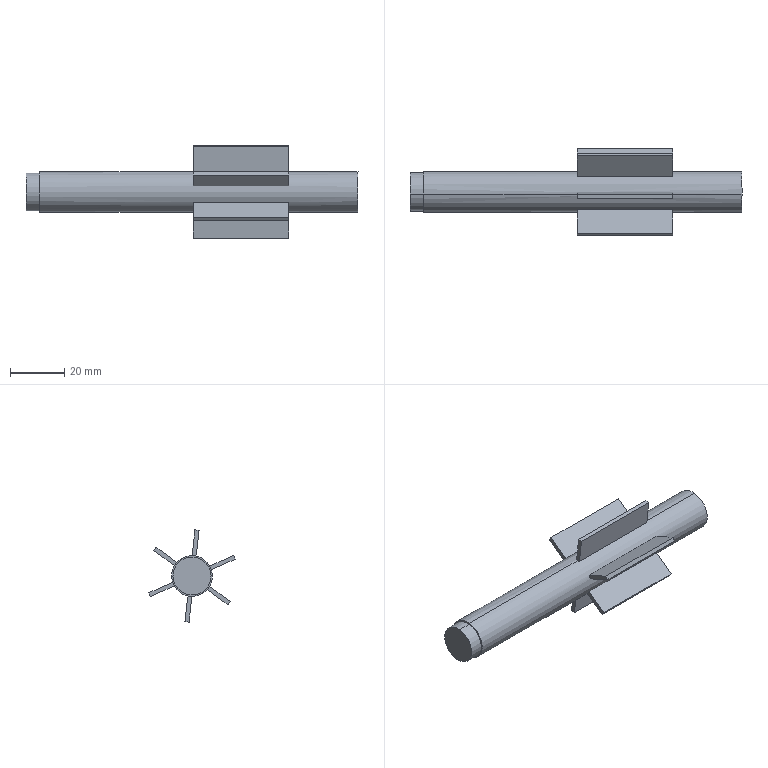Component | SolidWorks | HZ022-A001-E004-1 | 1 solid | 37 faces | box 122 x 31.71 x 33.96 mm | volume 24441 mm3 | plane 33 | cylinder 4 | commonest cylinder face diameters 13.99 x2 15 x2 | material S45C
STEP:
#1=COLOUR_RGB('',0.7922,0.8196,0.9333);
#2=FILL_AREA_STYLE_COLOUR('',#1);
#3=FILL_AREA_STYLE('',(#2));
#4=SURFACE_STYLE_FILL_AREA(#3);
#5=SURFACE_SIDE_STYLE('',(#4));
#6=SURFACE_STYLE_USAGE(.BOTH.,#5);
#7=PRESENTATION_STYLE_ASSIGNMENT((#6));
#8=CARTESIAN_POINT('',(-1.518,7.595,35.553));
#9=VERTEX_POINT('',#8);
#10=CARTESIAN_POINT('',(-1.518,7.535,36.101));
#11=VERTEX_POINT('',#10);
#12=CARTESIAN_POINT('',(-1.518,7.565,35.827));
#13=DIRECTION('',(1.,-0.,-0.));
#14=DIRECTION('',(-0.,0.108,-0.9942));
#15=AXIS2_PLACEMENT_3D('',#12,#13,#14);
#16=CIRCLE('',#15,0.2754);
#17=EDGE_CURVE('',#9,#11,#16,.T.);
#18=ORIENTED_EDGE('',*,*,#17,.F.);
#19=CARTESIAN_POINT('',(-1.715,7.595,35.553));
#20=VERTEX_POINT('',#19);
#21=CARTESIAN_POINT('',(-1.518,7.595,35.553));
#22=DIRECTION('',(-1.,0.,0.));
#23=VECTOR('',#22,39.37);
#24=LINE('',#21,#23);
#25=EDGE_CURVE('',#9,#20,#24,.T.);
#26=ORIENTED_EDGE('',*,*,#25,.T.);
#27=CARTESIAN_POINT('',(-1.715,7.535,36.101));
#28=VERTEX_POINT('',#27);
#29=CARTESIAN_POINT('',(-1.715,7.565,35.827));
#30=DIRECTION('',(-1.,0.,0.));
#31=DIRECTION('',(-0.,0.108,-0.9942));
#32=AXIS2_PLACEMENT_3D('',#29,#30,#31);
#33=CIRCLE('',#32,0.2754);
#34=EDGE_CURVE('',#28,#20,#33,.T.);
#35=ORIENTED_EDGE('',*,*,#34,.F.);
#36=CARTESIAN_POINT('',(-1.518,7.535,36.101));
#37=DIRECTION('',(-1.,0.,0.));
#38=VECTOR('',#37,39.37);
#39=LINE('',#36,#38);
#40=EDGE_CURVE('',#11,#28,#39,.T.);
#41=ORIENTED_EDGE('',*,*,#40,.F.);
#42=EDGE_LOOP('',(#18,#26,#35,#41));
#43=FACE_OUTER_BOUND('',#42,.T.);
#44=CARTESIAN_POINT('',(-1.518,7.565,35.827));
#45=DIRECTION('',(-1.,0.,0.));
#46=DIRECTION('',(0.,-0.108,0.9942));
#47=AXIS2_PLACEMENT_3D('',#44,#45,#46);
#48=CYLINDRICAL_SURFACE('',#47,0.2754);
#49=ADVANCED_FACE('',(#43),#48,.T.);
#50=CARTESIAN_POINT('',(2.084,7.785,36.024));
#51=VERTEX_POINT('',#50);
#52=CARTESIAN_POINT('',(2.084,7.82,35.976));
#53=VERTEX_POINT('',#52);
#54=CARTESIAN_POINT('',(2.084,7.565,35.827));
#55=DIRECTION('',(-1.,0.,0.));
#56=DIRECTION('',(0.,-0.108,0.9942));
#57=AXIS2_PLACEMENT_3D('',#54,#55,#56);
#58=CIRCLE('',#57,0.2953);
#59=EDGE_CURVE('',#51,#53,#58,.T.);
#60=ORIENTED_EDGE('',*,*,#59,.F.);
#61=CARTESIAN_POINT('',(0.7064,7.785,36.024));
#62=VERTEX_POINT('',#61);
#63=CARTESIAN_POINT('',(3.088,7.785,36.024));
#64=DIRECTION('',(-1.,0.,0.));
#65=VECTOR('',#64,39.37);
#66=LINE('',#63,#65);
#67=EDGE_CURVE('',#51,#62,#66,.T.);
#68=ORIENTED_EDGE('',*,*,#67,.T.);
#69=CARTESIAN_POINT('',(0.7064,7.82,35.976));
#70=VERTEX_POINT('',#69);
#71=CARTESIAN_POINT('',(0.7064,7.565,35.827));
#72=DIRECTION('',(-1.,0.,0.));
#73=DIRECTION('',(0.,-0.108,0.9942));
#74=AXIS2_PLACEMENT_3D('',#71,#72,#73);
#75=CIRCLE('',#74,0.2953);
#76=EDGE_CURVE('',#62,#70,#75,.T.);
#77=ORIENTED_EDGE('',*,*,#76,.T.);
#78=CARTESIAN_POINT('',(3.088,7.82,35.976));
#79=DIRECTION('',(1.,-0.,-0.));
#80=VECTOR('',#79,39.37);
#81=LINE('',#78,#80);
#82=EDGE_CURVE('',#70,#53,#81,.T.);
#83=ORIENTED_EDGE('',*,*,#82,.T.);
#84=EDGE_LOOP('',(#60,#68,#77,#83));
#85=FACE_BOUND('',#84,.T.);
#86=CARTESIAN_POINT('',(0.7064,7.846,35.735));
#87=VERTEX_POINT('',#86);
#88=CARTESIAN_POINT('',(0.7064,7.822,35.681));
#89=VERTEX_POINT('',#88);
#90=CARTESIAN_POINT('',(0.7064,7.565,35.827));
#91=DIRECTION('',(-1.,0.,0.));
#92=DIRECTION('',(0.,-0.108,0.9942));
#93=AXIS2_PLACEMENT_3D('',#90,#91,#92);
#94=CIRCLE('',#93,0.2953);
#95=EDGE_CURVE('',#87,#89,#94,.T.);
#96=ORIENTED_EDGE('',*,*,#95,.T.);
#97=CARTESIAN_POINT('',(2.084,7.822,35.681));
#98=VERTEX_POINT('',#97);
#99=CARTESIAN_POINT('',(3.088,7.822,35.681));
#100=DIRECTION('',(1.,-0.,-0.));
#101=VECTOR('',#100,39.37);
#102=LINE('',#99,#101);
#103=EDGE_CURVE('',#89,#98,#102,.T.);
#104=ORIENTED_EDGE('',*,*,#103,.T.);
#105=CARTESIAN_POINT('',(2.084,7.846,35.735));
#106=VERTEX_POINT('',#105);
#107=CARTESIAN_POINT('',(2.084,7.565,35.827));
#108=DIRECTION('',(-1.,0.,0.));
#109=DIRECTION('',(0.,-0.108,0.9942));
#110=AXIS2_PLACEMENT_3D('',#107,#108,#109);
#111=CIRCLE('',#110,0.2953);
#112=EDGE_CURVE('',#106,#98,#111,.T.);
#113=ORIENTED_EDGE('',*,*,#112,.F.);
#114=CARTESIAN_POINT('',(3.088,7.846,35.735));
#115=DIRECTION('',(1.,-0.,-0.));
#116=VECTOR('',#115,39.37);
#117=LINE('',#114,#116);
#118=EDGE_CURVE('',#87,#106,#117,.T.);
#119=ORIENTED_EDGE('',*,*,#118,.F.);
#120=EDGE_LOOP('',(#96,#104,#113,#119));
#121=FACE_BOUND('',#120,.T.);
#122=CARTESIAN_POINT('',(3.088,7.597,35.533));
#123=VERTEX_POINT('',#122);
#124=CARTESIAN_POINT('',(3.088,7.533,36.12));
#125=VERTEX_POINT('',#124);
#126=CARTESIAN_POINT('',(3.088,7.565,35.827));
#127=DIRECTION('',(1.,-0.,-0.));
#128=DIRECTION('',(-0.,0.108,-0.9942));
#129=AXIS2_PLACEMENT_3D('',#126,#127,#128);
#130=CIRCLE('',#129,0.2953);
#131=EDGE_CURVE('',#123,#125,#130,.T.);
#132=ORIENTED_EDGE('',*,*,#131,.F.);
#133=CARTESIAN_POINT('',(2.084,7.597,35.533));
#134=VERTEX_POINT('',#133);
#135=CARTESIAN_POINT('',(3.088,7.597,35.533));
#136=DIRECTION('',(-1.,0.,0.));
#137=VECTOR('',#136,39.37);
#138=LINE('',#135,#137);
#139=EDGE_CURVE('',#123,#134,#138,.T.);
#140=ORIENTED_EDGE('',*,*,#139,.T.);
#141=CARTESIAN_POINT('',(2.084,7.626,35.538));
#142=VERTEX_POINT('',#141);
#143=CARTESIAN_POINT('',(2.084,7.565,35.827));
#144=DIRECTION('',(-1.,0.,0.));
#145=DIRECTION('',(0.,-0.108,0.9942));
#146=AXIS2_PLACEMENT_3D('',#143,#144,#145);
#147=CIRCLE('',#146,0.2953);
#148=EDGE_CURVE('',#142,#134,#147,.T.);
#149=ORIENTED_EDGE('',*,*,#148,.F.);
#150=CARTESIAN_POINT('',(0.7064,7.626,35.538));
#151=VERTEX_POINT('',#150);
#152=CARTESIAN_POINT('',(3.088,7.626,35.538));
#153=DIRECTION('',(1.,-0.,-0.));
#154=VECTOR('',#153,39.37);
#155=LINE('',#152,#154);
#156=EDGE_CURVE('',#151,#142,#155,.T.);
#157=ORIENTED_EDGE('',*,*,#156,.F.);
#158=CARTESIAN_POINT('',(0.7064,7.597,35.533));
#159=VERTEX_POINT('',#158);
#160=CARTESIAN_POINT('',(0.7064,7.565,35.827));
#161=DIRECTION('',(-1.,0.,0.));
#162=DIRECTION('',(0.,-0.108,0.9942));
#163=AXIS2_PLACEMENT_3D('',#160,#161,#162);
#164=CIRCLE('',#163,0.2953);
#165=EDGE_CURVE('',#151,#159,#164,.T.);
#166=ORIENTED_EDGE('',*,*,#165,.T.);
#167=CARTESIAN_POINT('',(-1.518,7.597,35.533));
#168=VERTEX_POINT('',#167);
#169=CARTESIAN_POINT('',(3.088,7.597,35.533));
#170=DIRECTION('',(-1.,0.,0.));
#171=VECTOR('',#170,39.37);
#172=LINE('',#169,#171);
#173=EDGE_CURVE('',#159,#168,#172,.T.);
#174=ORIENTED_EDGE('',*,*,#173,.T.);
#175=CARTESIAN_POINT('',(-1.518,7.533,36.12));
#176=VERTEX_POINT('',#175);
#177=CARTESIAN_POINT('',(-1.518,7.565,35.827));
#178=DIRECTION('',(1.,-0.,-0.));
#179=DIRECTION('',(-0.,0.108,-0.9942));
#180=AXIS2_PLACEMENT_3D('',#177,#178,#179);
#181=CIRCLE('',#180,0.2953);
#182=EDGE_CURVE('',#168,#176,#181,.T.);
#183=ORIENTED_EDGE('',*,*,#182,.T.);
#184=CARTESIAN_POINT('',(0.7064,7.533,36.12));
#185=VERTEX_POINT('',#184);
#186=CARTESIAN_POINT('',(3.088,7.533,36.12));
#187=DIRECTION('',(-1.,0.,0.));
#188=VECTOR('',#187,39.37);
#189=LINE('',#186,#188);
#190=EDGE_CURVE('',#185,#176,#189,.T.);
#191=ORIENTED_EDGE('',*,*,#190,.F.);
#192=CARTESIAN_POINT('',(0.7064,7.563,36.122));
#193=VERTEX_POINT('',#192);
#194=CARTESIAN_POINT('',(0.7064,7.565,35.827));
#195=DIRECTION('',(-1.,0.,0.));
#196=DIRECTION('',(0.,-0.108,0.9942));
#197=AXIS2_PLACEMENT_3D('',#194,#195,#196);
#198=CIRCLE('',#197,0.2953);
#199=EDGE_CURVE('',#185,#193,#198,.T.);
#200=ORIENTED_EDGE('',*,*,#199,.T.);
#201=CARTESIAN_POINT('',(2.084,7.563,36.122));
#202=VERTEX_POINT('',#201);
#203=CARTESIAN_POINT('',(3.088,7.563,36.122));
#204=DIRECTION('',(1.,-0.,-0.));
#205=VECTOR('',#204,39.37);
#206=LINE('',#203,#205);
#207=EDGE_CURVE('',#193,#202,#206,.T.);
#208=ORIENTED_EDGE('',*,*,#207,.T.);
#209=CARTESIAN_POINT('',(2.084,7.533,36.12));
#210=VERTEX_POINT('',#209);
#211=CARTESIAN_POINT('',(2.084,7.565,35.827));
#212=DIRECTION('',(-1.,0.,0.));
#213=DIRECTION('',(0.,-0.108,0.9942));
#214=AXIS2_PLACEMENT_3D('',#211,#212,#213);
#215=CIRCLE('',#214,0.2953);
#216=EDGE_CURVE('',#210,#202,#215,.T.);
#217=ORIENTED_EDGE('',*,*,#216,.F.);
#218=CARTESIAN_POINT('',(3.088,7.533,36.12));
#219=DIRECTION('',(-1.,0.,0.));
#220=VECTOR('',#219,39.37);
#221=LINE('',#218,#220);
#222=EDGE_CURVE('',#125,#210,#221,.T.);
#223=ORIENTED_EDGE('',*,*,#222,.F.);
#224=EDGE_LOOP('',(#132,#140,#149,#157,#166,#174,#183,#191,#200,#208,#217,#223));
#225=FACE_OUTER_BOUND('',#224,.T.);
#226=CARTESIAN_POINT('',(3.088,7.565,35.827));
#227=DIRECTION('',(-1.,0.,0.));
#228=DIRECTION('',(0.,-0.108,0.9942));
#229=AXIS2_PLACEMENT_3D('',#226,#227,#228);
#230=CYLINDRICAL_SURFACE('',#229,0.2953);
#231=ADVANCED_FACE('',(#85,#121,#225),#230,.T.);
#232=ORIENTED_EDGE('',*,*,#139,.F.);
#233=CARTESIAN_POINT('',(3.088,7.565,35.827));
#234=DIRECTION('',(1.,-0.,-0.));
#235=DIRECTION('',(-0.,0.108,-0.9942));
#236=AXIS2_PLACEMENT_3D('',#233,#234,#235);
#237=CIRCLE('',#236,0.2953);
#238=EDGE_CURVE('',#125,#123,#237,.T.);
#239=ORIENTED_EDGE('',*,*,#238,.F.);
#240=ORIENTED_EDGE('',*,*,#222,.T.);
#241=CARTESIAN_POINT('',(2.084,7.504,36.116));
#242=VERTEX_POINT('',#241);
#243=CARTESIAN_POINT('',(2.084,7.565,35.827));
#244=DIRECTION('',(-1.,0.,0.));
#245=DIRECTION('',(0.,-0.108,0.9942));
#246=AXIS2_PLACEMENT_3D('',#243,#244,#245);
#247=CIRCLE('',#246,0.2953);
#248=EDGE_CURVE('',#242,#210,#247,.T.);
#249=ORIENTED_EDGE('',*,*,#248,.F.);
#250=CARTESIAN_POINT('',(0.7064,7.504,36.116));
#251=VERTEX_POINT('',#250);
#252=CARTESIAN_POINT('',(3.088,7.504,36.116));
#253=DIRECTION('',(1.,-0.,-0.));
#254=VECTOR('',#253,39.37);
#255=LINE('',#252,#254);
#256=EDGE_CURVE('',#251,#242,#255,.T.);
#257=ORIENTED_EDGE('',*,*,#256,.F.);
#258=CARTESIAN_POINT('',(0.7064,7.565,35.827));
#259=DIRECTION('',(-1.,0.,0.));
#260=DIRECTION('',(0.,-0.108,0.9942));
#261=AXIS2_PLACEMENT_3D('',#258,#259,#260);
#262=CIRCLE('',#261,0.2953);
#263=EDGE_CURVE('',#251,#185,#262,.T.);
#264=ORIENTED_EDGE('',*,*,#263,.T.);
#265=ORIENTED_EDGE('',*,*,#190,.T.);
#266=CARTESIAN_POINT('',(-1.518,7.565,35.827));
#267=DIRECTION('',(1.,-0.,-0.));
#268=DIRECTION('',(-0.,0.108,-0.9942));
#269=AXIS2_PLACEMENT_3D('',#266,#267,#268);
#270=CIRCLE('',#269,0.2953);
#271=EDGE_CURVE('',#176,#168,#270,.T.);
#272=ORIENTED_EDGE('',*,*,#271,.T.);
#273=ORIENTED_EDGE('',*,*,#173,.F.);
#274=CARTESIAN_POINT('',(0.7064,7.567,35.532));
#275=VERTEX_POINT('',#274);
#276=CARTESIAN_POINT('',(0.7064,7.565,35.827));
#277=DIRECTION('',(-1.,0.,0.));
#278=DIRECTION('',(0.,-0.108,0.9942));
#279=AXIS2_PLACEMENT_3D('',#276,#277,#278);
#280=CIRCLE('',#279,0.2953);
#281=EDGE_CURVE('',#159,#275,#280,.T.);
#282=ORIENTED_EDGE('',*,*,#281,.T.);
#283=CARTESIAN_POINT('',(2.084,7.567,35.532));
#284=VERTEX_POINT('',#283);
#285=CARTESIAN_POINT('',(3.088,7.567,35.532));
#286=DIRECTION('',(1.,-0.,-0.));
#287=VECTOR('',#286,39.37);
#288=LINE('',#285,#287);
#289=EDGE_CURVE('',#275,#284,#288,.T.);
#290=ORIENTED_EDGE('',*,*,#289,.T.);
#291=CARTESIAN_POINT('',(2.084,7.565,35.827));
#292=DIRECTION('',(-1.,0.,0.));
#293=DIRECTION('',(0.,-0.108,0.9942));
#294=AXIS2_PLACEMENT_3D('',#291,#292,#293);
#295=CIRCLE('',#294,0.2953);
#296=EDGE_CURVE('',#134,#284,#295,.T.);
#297=ORIENTED_EDGE('',*,*,#296,.F.);
#298=EDGE_LOOP('',(#232,#239,#240,#249,#257,#264,#265,#272,#273,#282,#290,#297));
#299=FACE_OUTER_BOUND('',#298,.T.);
#300=CARTESIAN_POINT('',(0.7064,7.284,35.918));
#301=VERTEX_POINT('',#300);
#302=CARTESIAN_POINT('',(2.084,7.284,35.918));
#303=VERTEX_POINT('',#302);
#304=CARTESIAN_POINT('',(3.088,7.284,35.918));
#305=DIRECTION('',(1.,-0.,-0.));
#306=VECTOR('',#305,39.37);
#307=LINE('',#304,#306);
#308=EDGE_CURVE('',#301,#303,#307,.T.);
#309=ORIENTED_EDGE('',*,*,#308,.F.);
#310=CARTESIAN_POINT('',(0.7064,7.308,35.972));
#311=VERTEX_POINT('',#310);
#312=CARTESIAN_POINT('',(0.7064,7.565,35.827));
#313=DIRECTION('',(-1.,0.,0.));
#314=DIRECTION('',(0.,-0.108,0.9942));
#315=AXIS2_PLACEMENT_3D('',#312,#313,#314);
#316=CIRCLE('',#315,0.2953);
#317=EDGE_CURVE('',#301,#311,#316,.T.);
#318=ORIENTED_EDGE('',*,*,#317,.T.);
#319=CARTESIAN_POINT('',(2.084,7.308,35.972));
#320=VERTEX_POINT('',#319);
#321=CARTESIAN_POINT('',(3.088,7.308,35.972));
#322=DIRECTION('',(1.,-0.,-0.));
#323=VECTOR('',#322,39.37);
#324=LINE('',#321,#323);
#325=EDGE_CURVE('',#311,#320,#324,.T.);
#326=ORIENTED_EDGE('',*,*,#325,.T.);
#327=CARTESIAN_POINT('',(2.084,7.565,35.827));
#328=DIRECTION('',(-1.,0.,0.));
#329=DIRECTION('',(0.,-0.108,0.9942));
#330=AXIS2_PLACEMENT_3D('',#327,#328,#329);
#331=CIRCLE('',#330,0.2953);
#332=EDGE_CURVE('',#303,#320,#331,.T.);
#333=ORIENTED_EDGE('',*,*,#332,.F.);
#334=EDGE_LOOP('',(#309,#318,#326,#333));
#335=FACE_BOUND('',#334,.T.);
#336=CARTESIAN_POINT('',(0.7064,7.345,35.629));
#337=VERTEX_POINT('',#336);
#338=CARTESIAN_POINT('',(0.7064,7.311,35.677));
#339=VERTEX_POINT('',#338);
#340=CARTESIAN_POINT('',(0.7064,7.565,35.827));
#341=DIRECTION('',(-1.,0.,0.));
#342=DIRECTION('',(0.,-0.108,0.9942));
#343=AXIS2_PLACEMENT_3D('',#340,#341,#342);
#344=CIRCLE('',#343,0.2953);
#345=EDGE_CURVE('',#337,#339,#344,.T.);
#346=ORIENTED_EDGE('',*,*,#345,.T.);
#347=CARTESIAN_POINT('',(2.084,7.311,35.677));
#348=VERTEX_POINT('',#347);
#349=CARTESIAN_POINT('',(3.088,7.311,35.677));
#350=DIRECTION('',(1.,-0.,-0.));
#351=VECTOR('',#350,39.37);
#352=LINE('',#349,#351);
#353=EDGE_CURVE('',#339,#348,#352,.T.);
#354=ORIENTED_EDGE('',*,*,#353,.T.);
#355=CARTESIAN_POINT('',(2.084,7.345,35.629));
#356=VERTEX_POINT('',#355);
#357=CARTESIAN_POINT('',(2.084,7.565,35.827));
#358=DIRECTION('',(-1.,0.,0.));
#359=DIRECTION('',(0.,-0.108,0.9942));
#360=AXIS2_PLACEMENT_3D('',#357,#358,#359);
#361=CIRCLE('',#360,0.2953);
#362=EDGE_CURVE('',#356,#348,#361,.T.);
#363=ORIENTED_EDGE('',*,*,#362,.F.);
#364=CARTESIAN_POINT('',(3.088,7.345,35.629));
#365=DIRECTION('',(1.,-0.,-0.));
#366=VECTOR('',#365,39.37);
#367=LINE('',#364,#366);
#368=EDGE_CURVE('',#337,#356,#367,.T.);
#369=ORIENTED_EDGE('',*,*,#368,.F.);
#370=EDGE_LOOP('',(#346,#354,#363,#369));
#371=FACE_BOUND('',#370,.T.);
#372=CARTESIAN_POINT('',(3.088,7.565,35.827));
#373=DIRECTION('',(-1.,0.,0.));
#374=DIRECTION('',(0.,-0.108,0.9942));
#375=AXIS2_PLACEMENT_3D('',#372,#373,#374);
#376=CYLINDRICAL_SURFACE('',#375,0.2953);
#377=ADVANCED_FACE('',(#299,#335,#371),#376,.T.);
#378=ORIENTED_EDGE('',*,*,#238,.T.);
#379=ORIENTED_EDGE('',*,*,#131,.T.);
#380=EDGE_LOOP('',(#378,#379));
#381=FACE_OUTER_BOUND('',#380,.T.);
#382=CARTESIAN_POINT('',(3.088,7.565,35.827));
#383=DIRECTION('',(1.,-0.,-0.));
#384=DIRECTION('',(-0.,0.108,-0.9942));
#385=AXIS2_PLACEMENT_3D('',#382,#383,#384);
#386=PLANE('',#385);
#387=ADVANCED_FACE('',(#381),#386,.T.);
#388=ORIENTED_EDGE('',*,*,#207,.F.);
#389=CARTESIAN_POINT('',(0.7064,7.522,36.495));
#390=VERTEX_POINT('',#389);
#391=CARTESIAN_POINT('',(0.7064,7.594,35.83));
#392=DIRECTION('',(0.,-0.108,0.9942));
#393=VECTOR('',#392,39.37);
#394=LINE('',#391,#393);
#395=EDGE_CURVE('',#193,#390,#394,.T.);
#396=ORIENTED_EDGE('',*,*,#395,.T.);
#397=CARTESIAN_POINT('',(2.084,7.522,36.495));
#398=VERTEX_POINT('',#397);
#399=CARTESIAN_POINT('',(0.7064,7.522,36.495));
#400=DIRECTION('',(1.,-0.,-0.));
#401=VECTOR('',#400,39.37);
#402=LINE('',#399,#401);
#403=EDGE_CURVE('',#390,#398,#402,.T.);
#404=ORIENTED_EDGE('',*,*,#403,.T.);
#405=CARTESIAN_POINT('',(2.084,7.594,35.83));
#406=DIRECTION('',(0.,-0.108,0.9942));
#407=VECTOR('',#406,39.37);
#408=LINE('',#405,#407);
#409=EDGE_CURVE('',#202,#398,#408,.T.);
#410=ORIENTED_EDGE('',*,*,#409,.F.);
#411=EDGE_LOOP('',(#388,#396,#404,#410));
#412=FACE_OUTER_BOUND('',#411,.T.);
#413=CARTESIAN_POINT('',(0.7064,7.594,35.83));
#414=DIRECTION('',(0.,0.9942,0.108));
#415=DIRECTION('',(0.,-0.108,0.9942));
#416=AXIS2_PLACEMENT_3D('',#413,#414,#415);
#417=PLANE('',#416);
#418=ADVANCED_FACE('',(#412),#417,.T.);
#419=CARTESIAN_POINT('',(0.7064,7.463,36.489));
#420=VERTEX_POINT('',#419);
#421=CARTESIAN_POINT('',(0.7064,7.536,35.824));
#422=DIRECTION('',(0.,-0.108,0.9942));
#423=VECTOR('',#422,39.37);
#424=LINE('',#421,#423);
#425=EDGE_CURVE('',#251,#420,#424,.T.);
#426=ORIENTED_EDGE('',*,*,#425,.F.);
#427=ORIENTED_EDGE('',*,*,#256,.T.);
#428=CARTESIAN_POINT('',(2.084,7.463,36.489));
#429=VERTEX_POINT('',#428);
#430=CARTESIAN_POINT('',(2.084,7.536,35.824));
#431=DIRECTION('',(0.,-0.108,0.9942));
#432=VECTOR('',#431,39.37);
#433=LINE('',#430,#432);
#434=EDGE_CURVE('',#242,#429,#433,.T.);
#435=ORIENTED_EDGE('',*,*,#434,.T.);
#436=CARTESIAN_POINT('',(0.7064,7.463,36.489));
#437=DIRECTION('',(1.,-0.,-0.));
#438=VECTOR('',#437,39.37);
#439=LINE('',#436,#438);
#440=EDGE_CURVE('',#420,#429,#439,.T.);
#441=ORIENTED_EDGE('',*,*,#440,.F.);
#442=EDGE_LOOP('',(#426,#427,#435,#441));
#443=FACE_OUTER_BOUND('',#442,.T.);
#444=CARTESIAN_POINT('',(0.7064,7.536,35.824));
#445=DIRECTION('',(0.,0.9942,0.108));
#446=DIRECTION('',(0.,-0.108,0.9942));
#447=AXIS2_PLACEMENT_3D('',#444,#445,#446);
#448=PLANE('',#447);
#449=ADVANCED_FACE('',(#443),#448,.F.);
#450=CARTESIAN_POINT('',(2.084,7.463,36.489));
#451=DIRECTION('',(0.,0.9942,0.108));
#452=VECTOR('',#451,39.37);
#453=LINE('',#450,#452);
#454=EDGE_CURVE('',#429,#398,#453,.T.);
#455=ORIENTED_EDGE('',*,*,#454,.T.);
#456=ORIENTED_EDGE('',*,*,#403,.F.);
#457=CARTESIAN_POINT('',(0.7064,7.463,36.489));
#458=DIRECTION('',(0.,0.9942,0.108));
#459=VECTOR('',#458,39.37);
#460=LINE('',#457,#459);
#461=EDGE_CURVE('',#420,#390,#460,.T.);
#462=ORIENTED_EDGE('',*,*,#461,.F.);
#463=ORIENTED_EDGE('',*,*,#440,.T.);
#464=EDGE_LOOP('',(#455,#456,#462,#463));
#465=FACE_OUTER_BOUND('',#464,.T.);
#466=CARTESIAN_POINT('',(0.7064,7.463,36.489));
#467=DIRECTION('',(-0.,0.108,-0.9942));
#468=DIRECTION('',(0.,0.9942,0.108));
#469=AXIS2_PLACEMENT_3D('',#466,#467,#468);
#470=PLANE('',#469);
#471=ADVANCED_FACE('',(#465),#470,.F.);
#472=ORIENTED_EDGE('',*,*,#263,.F.);
#473=ORIENTED_EDGE('',*,*,#425,.T.);
#474=ORIENTED_EDGE('',*,*,#461,.T.);
#475=ORIENTED_EDGE('',*,*,#395,.F.);
#476=ORIENTED_EDGE('',*,*,#199,.F.);
#477=EDGE_LOOP('',(#472,#473,#474,#475,#476));
#478=FACE_OUTER_BOUND('',#477,.T.);
#479=CARTESIAN_POINT('',(0.7064,7.565,35.827));
#480=DIRECTION('',(-1.,0.,0.));
#481=DIRECTION('',(-0.,-0.9942,-0.108));
#482=AXIS2_PLACEMENT_3D('',#479,#480,#481);
#483=PLANE('',#482);
#484=ADVANCED_FACE('',(#478),#483,.T.);
#485=ORIENTED_EDGE('',*,*,#434,.F.);
#486=ORIENTED_EDGE('',*,*,#248,.T.);
#487=ORIENTED_EDGE('',*,*,#216,.T.);
#488=ORIENTED_EDGE('',*,*,#409,.T.);
#489=ORIENTED_EDGE('',*,*,#454,.F.);
#490=EDGE_LOOP('',(#485,#486,#487,#488,#489));
#491=FACE_OUTER_BOUND('',#490,.T.);
#492=CARTESIAN_POINT('',(2.084,7.565,35.827));
#493=DIRECTION('',(-1.,0.,0.));
#494=DIRECTION('',(-0.,-0.9942,-0.108));
#495=AXIS2_PLACEMENT_3D('',#492,#493,#494);
#496=PLANE('',#495);
#497=ADVANCED_FACE('',(#491),#496,.F.);
#498=CARTESIAN_POINT('',(2.084,8.088,36.246));
#499=VERTEX_POINT('',#498);
#500=CARTESIAN_POINT('',(2.084,8.123,36.198));
#501=VERTEX_POINT('',#500);
#502=CARTESIAN_POINT('',(2.084,8.088,36.246));
#503=DIRECTION('',(-0.,0.5906,-0.807));
#504=VECTOR('',#503,39.37);
#505=LINE('',#502,#504);
#506=EDGE_CURVE('',#499,#501,#505,.T.);
#507=ORIENTED_EDGE('',*,*,#506,.T.);
#508=CARTESIAN_POINT('',(0.7064,8.123,36.198));
#509=VERTEX_POINT('',#508);
#510=CARTESIAN_POINT('',(0.7064,8.123,36.198));
#511=DIRECTION('',(1.,-0.,-0.));
#512=VECTOR('',#511,39.37);
#513=LINE('',#510,#512);
#514=EDGE_CURVE('',#509,#501,#513,.T.);
#515=ORIENTED_EDGE('',*,*,#514,.F.);
#516=CARTESIAN_POINT('',(0.7064,8.088,36.246));
#517=VERTEX_POINT('',#516);
#518=CARTESIAN_POINT('',(0.7064,8.088,36.246));
#519=DIRECTION('',(-0.,0.5906,-0.807));
#520=VECTOR('',#519,39.37);
#521=LINE('',#518,#520);
#522=EDGE_CURVE('',#517,#509,#521,.T.);
#523=ORIENTED_EDGE('',*,*,#522,.F.);
#524=CARTESIAN_POINT('',(0.7064,8.088,36.246));
#525=DIRECTION('',(1.,-0.,-0.));
#526=VECTOR('',#525,39.37);
#527=LINE('',#524,#526);
#528=EDGE_CURVE('',#517,#499,#527,.T.);
#529=ORIENTED_EDGE('',*,*,#528,.T.);
#530=EDGE_LOOP('',(#507,#515,#523,#529));
#531=FACE_OUTER_BOUND('',#530,.T.);
#532=CARTESIAN_POINT('',(0.7064,8.088,36.246));
#533=DIRECTION('',(-0.,-0.807,-0.5906));
#534=DIRECTION('',(-0.,0.5906,-0.807));
#535=AXIS2_PLACEMENT_3D('',#532,#533,#534);
#536=PLANE('',#535);
#537=ADVANCED_FACE('',(#531),#536,.F.);
#538=ORIENTED_EDGE('',*,*,#82,.F.);
#539=CARTESIAN_POINT('',(0.7064,7.582,35.803));
#540=DIRECTION('',(0.,0.807,0.5906));
#541=VECTOR('',#540,39.37);
#542=LINE('',#539,#541);
#543=EDGE_CURVE('',#70,#509,#542,.T.);
#544=ORIENTED_EDGE('',*,*,#543,.T.);
#545=ORIENTED_EDGE('',*,*,#514,.T.);
#546=CARTESIAN_POINT('',(2.084,7.582,35.803));
#547=DIRECTION('',(0.,0.807,0.5906));
#548=VECTOR('',#547,39.37);
#549=LINE('',#546,#548);
#550=EDGE_CURVE('',#53,#501,#549,.T.);
#551=ORIENTED_EDGE('',*,*,#550,.F.);
#552=EDGE_LOOP('',(#538,#544,#545,#551));
#553=FACE_OUTER_BOUND('',#552,.T.);
#554=CARTESIAN_POINT('',(0.7064,7.582,35.803));
#555=DIRECTION('',(-0.,0.5906,-0.807));
#556=DIRECTION('',(0.,0.807,0.5906));
#557=AXIS2_PLACEMENT_3D('',#554,#555,#556);
#558=PLANE('',#557);
#559=ADVANCED_FACE('',(#553),#558,.T.);
#560=ORIENTED_EDGE('',*,*,#67,.F.);
#561=CARTESIAN_POINT('',(2.084,7.548,35.851));
#562=DIRECTION('',(-0.,-0.807,-0.5906));
#563=VECTOR('',#562,39.37);
#564=LINE('',#561,#563);
#565=EDGE_CURVE('',#499,#51,#564,.T.);
#566=ORIENTED_EDGE('',*,*,#565,.F.);
#567=ORIENTED_EDGE('',*,*,#528,.F.);
#568=CARTESIAN_POINT('',(0.7064,7.548,35.851));
#569=DIRECTION('',(-0.,-0.807,-0.5906));
#570=VECTOR('',#569,39.37);
#571=LINE('',#568,#570);
#572=EDGE_CURVE('',#517,#62,#571,.T.);
#573=ORIENTED_EDGE('',*,*,#572,.T.);
#574=EDGE_LOOP('',(#560,#566,#567,#573));
#575=FACE_OUTER_BOUND('',#574,.T.);
#576=CARTESIAN_POINT('',(0.7064,7.548,35.851));
#577=DIRECTION('',(0.,-0.5906,0.807));
#578=DIRECTION('',(-0.,-0.807,-0.5906));
#579=AXIS2_PLACEMENT_3D('',#576,#577,#578);
#580=PLANE('',#579);
#581=ADVANCED_FACE('',(#575),#580,.T.);
#582=ORIENTED_EDGE('',*,*,#565,.T.);
#583=ORIENTED_EDGE('',*,*,#59,.T.);
#584=ORIENTED_EDGE('',*,*,#550,.T.);
#585=ORIENTED_EDGE('',*,*,#506,.F.);
#586=EDGE_LOOP('',(#582,#583,#584,#585));
#587=FACE_OUTER_BOUND('',#586,.T.);
#588=CARTESIAN_POINT('',(2.084,7.565,35.827));
#589=DIRECTION('',(-1.,0.,0.));
#590=DIRECTION('',(-0.,-0.4035,-0.915));
#591=AXIS2_PLACEMENT_3D('',#588,#589,#590);
#592=PLANE('',#591);
#593=ADVANCED_FACE('',(#587),#592,.F.);
#594=ORIENTED_EDGE('',*,*,#76,.F.);
#595=ORIENTED_EDGE('',*,*,#572,.F.);
#596=ORIENTED_EDGE('',*,*,#522,.T.);
#597=ORIENTED_EDGE('',*,*,#543,.F.);
#598=EDGE_LOOP('',(#594,#595,#596,#597));
#599=FACE_OUTER_BOUND('',#598,.T.);
#600=CARTESIAN_POINT('',(0.7064,7.565,35.827));
#601=DIRECTION('',(-1.,0.,0.));
#602=DIRECTION('',(-0.,-0.4035,-0.915));
#603=AXIS2_PLACEMENT_3D('',#600,#601,#602);
#604=PLANE('',#603);
#605=ADVANCED_FACE('',(#599),#604,.T.);
#606=CARTESIAN_POINT('',(2.084,8.189,35.584));
#607=VERTEX_POINT('',#606);
#608=CARTESIAN_POINT('',(2.084,8.165,35.53));
#609=VERTEX_POINT('',#608);
#610=CARTESIAN_POINT('',(2.084,8.189,35.584));
#611=DIRECTION('',(-0.,-0.4035,-0.915));
#612=VECTOR('',#611,39.37);
#613=LINE('',#610,#612);
#614=EDGE_CURVE('',#607,#609,#613,.T.);
#615=ORIENTED_EDGE('',*,*,#614,.T.);
#616=CARTESIAN_POINT('',(0.7064,8.165,35.53));
#617=VERTEX_POINT('',#616);
#618=CARTESIAN_POINT('',(0.7064,8.165,35.53));
#619=DIRECTION('',(1.,-0.,-0.));
#620=VECTOR('',#619,39.37);
#621=LINE('',#618,#620);
#622=EDGE_CURVE('',#617,#609,#621,.T.);
#623=ORIENTED_EDGE('',*,*,#622,.F.);
#624=CARTESIAN_POINT('',(0.7064,8.189,35.584));
#625=VERTEX_POINT('',#624);
#626=CARTESIAN_POINT('',(0.7064,8.189,35.584));
#627=DIRECTION('',(-0.,-0.4035,-0.915));
#628=VECTOR('',#627,39.37);
#629=LINE('',#626,#628);
#630=EDGE_CURVE('',#625,#617,#629,.T.);
#631=ORIENTED_EDGE('',*,*,#630,.F.);
#632=CARTESIAN_POINT('',(0.7064,8.189,35.584));
#633=DIRECTION('',(1.,-0.,-0.));
#634=VECTOR('',#633,39.37);
#635=LINE('',#632,#634);
#636=EDGE_CURVE('',#625,#607,#635,.T.);
#637=ORIENTED_EDGE('',*,*,#636,.T.);
#638=EDGE_LOOP('',(#615,#623,#631,#637));
#639=FACE_OUTER_BOUND('',#638,.T.);
#640=CARTESIAN_POINT('',(0.7064,8.189,35.584));
#641=DIRECTION('',(0.,-0.915,0.4035));
#642=DIRECTION('',(-0.,-0.4035,-0.915));
#643=AXIS2_PLACEMENT_3D('',#640,#641,#642);
#644=PLANE('',#643);
#645=ADVANCED_FACE('',(#639),#644,.F.);
#646=ORIENTED_EDGE('',*,*,#103,.F.);
#647=CARTESIAN_POINT('',(0.7064,7.553,35.8));
#648=DIRECTION('',(-0.,0.915,-0.4035));
#649=VECTOR('',#648,39.37);
#650=LINE('',#647,#649);
#651=EDGE_CURVE('',#89,#617,#650,.T.);
#652=ORIENTED_EDGE('',*,*,#651,.T.);
#653=ORIENTED_EDGE('',*,*,#622,.T.);
#654=CARTESIAN_POINT('',(2.084,7.553,35.8));
#655=DIRECTION('',(-0.,0.915,-0.4035));
#656=VECTOR('',#655,39.37);
#657=LINE('',#654,#656);
#658=EDGE_CURVE('',#98,#609,#657,.T.);
#659=ORIENTED_EDGE('',*,*,#658,.F.);
#660=EDGE_LOOP('',(#646,#652,#653,#659));
#661=FACE_OUTER_BOUND('',#660,.T.);
#662=CARTESIAN_POINT('',(0.7064,7.553,35.8));
#663=DIRECTION('',(-0.,-0.4035,-0.915));
#664=DIRECTION('',(-0.,0.915,-0.4035));
#665=AXIS2_PLACEMENT_3D('',#662,#663,#664);
#666=PLANE('',#665);
#667=ADVANCED_FACE('',(#661),#666,.T.);
#668=CARTESIAN_POINT('',(0.7064,7.577,35.854));
#669=DIRECTION('',(-0.,0.915,-0.4035));
#670=VECTOR('',#669,39.37);
#671=LINE('',#668,#670);
#672=EDGE_CURVE('',#87,#625,#671,.T.);
#673=ORIENTED_EDGE('',*,*,#672,.F.);
#674=ORIENTED_EDGE('',*,*,#118,.T.);
#675=CARTESIAN_POINT('',(2.084,7.577,35.854));
#676=DIRECTION('',(-0.,0.915,-0.4035));
#677=VECTOR('',#676,39.37);
#678=LINE('',#675,#677);
#679=EDGE_CURVE('',#106,#607,#678,.T.);
#680=ORIENTED_EDGE('',*,*,#679,.T.);
#681=ORIENTED_EDGE('',*,*,#636,.F.);
#682=EDGE_LOOP('',(#673,#674,#680,#681));
#683=FACE_OUTER_BOUND('',#682,.T.);
#684=CARTESIAN_POINT('',(0.7064,7.577,35.854));
#685=DIRECTION('',(-0.,-0.4035,-0.915));
#686=DIRECTION('',(-0.,0.915,-0.4035));
#687=AXIS2_PLACEMENT_3D('',#684,#685,#686);
#688=PLANE('',#687);
#689=ADVANCED_FACE('',(#683),#688,.F.);
#690=ORIENTED_EDGE('',*,*,#679,.F.);
#691=ORIENTED_EDGE('',*,*,#112,.T.);
#692=ORIENTED_EDGE('',*,*,#658,.T.);
#693=ORIENTED_EDGE('',*,*,#614,.F.);
#694=EDGE_LOOP('',(#690,#691,#692,#693));
#695=FACE_OUTER_BOUND('',#694,.T.);
#696=CARTESIAN_POINT('',(2.084,7.565,35.827));
#697=DIRECTION('',(-1.,0.,0.));
#698=DIRECTION('',(-0.,-0.4035,-0.915));
#699=AXIS2_PLACEMENT_3D('',#696,#697,#698);
#700=PLANE('',#699);
#701=ADVANCED_FACE('',(#695),#700,.F.);
#702=ORIENTED_EDGE('',*,*,#95,.F.);
#703=ORIENTED_EDGE('',*,*,#672,.T.);
#704=ORIENTED_EDGE('',*,*,#630,.T.);
#705=ORIENTED_EDGE('',*,*,#651,.F.);
#706=EDGE_LOOP('',(#702,#703,#704,#705));
#707=FACE_OUTER_BOUND('',#706,.T.);
#708=CARTESIAN_POINT('',(0.7064,7.565,35.827));
#709=DIRECTION('',(-1.,0.,0.));
#710=DIRECTION('',(-0.,-0.4035,-0.915));
#711=AXIS2_PLACEMENT_3D('',#708,#709,#710);
#712=PLANE('',#711);
#713=ADVANCED_FACE('',(#707),#712,.T.);
#714=CARTESIAN_POINT('',(2.084,7.667,35.165));
#715=VERTEX_POINT('',#714);
#716=CARTESIAN_POINT('',(2.084,7.608,35.158));
#717=VERTEX_POINT('',#716);
#718=CARTESIAN_POINT('',(2.084,7.667,35.165));
#719=DIRECTION('',(-0.,-0.9942,-0.108));
#720=VECTOR('',#719,39.37);
#721=LINE('',#718,#720);
#722=EDGE_CURVE('',#715,#717,#721,.T.);
#723=ORIENTED_EDGE('',*,*,#722,.T.);
#724=CARTESIAN_POINT('',(0.7064,7.608,35.158));
#725=VERTEX_POINT('',#724);
#726=CARTESIAN_POINT('',(0.7064,7.608,35.158));
#727=DIRECTION('',(1.,-0.,-0.));
#728=VECTOR('',#727,39.37);
#729=LINE('',#726,#728);
#730=EDGE_CURVE('',#725,#717,#729,.T.);
#731=ORIENTED_EDGE('',*,*,#730,.F.);
#732=CARTESIAN_POINT('',(0.7064,7.667,35.165));
#733=VERTEX_POINT('',#732);
#734=CARTESIAN_POINT('',(0.7064,7.667,35.165));
#735=DIRECTION('',(-0.,-0.9942,-0.108));
#736=VECTOR('',#735,39.37);
#737=LINE('',#734,#736);
#738=EDGE_CURVE('',#733,#725,#737,.T.);
#739=ORIENTED_EDGE('',*,*,#738,.F.);
#740=CARTESIAN_POINT('',(0.7064,7.667,35.165));
#741=DIRECTION('',(1.,-0.,-0.));
#742=VECTOR('',#741,39.37);
#743=LINE('',#740,#742);
#744=EDGE_CURVE('',#733,#715,#743,.T.);
#745=ORIENTED_EDGE('',*,*,#744,.T.);
#746=EDGE_LOOP('',(#723,#731,#739,#745));
#747=FACE_OUTER_BOUND('',#746,.T.);
#748=CARTESIAN_POINT('',(0.7064,7.667,35.165));
#749=DIRECTION('',(0.,-0.108,0.9942));
#750=DIRECTION('',(-0.,-0.9942,-0.108));
#751=AXIS2_PLACEMENT_3D('',#748,#749,#750);
#752=PLANE('',#751);
#753=ADVANCED_FACE('',(#747),#752,.F.);
#754=ORIENTED_EDGE('',*,*,#289,.F.);
#755=CARTESIAN_POINT('',(0.7064,7.536,35.824));
#756=DIRECTION('',(-0.,0.108,-0.9942));
#757=VECTOR('',#756,39.37);
#758=LINE('',#755,#757);
#759=EDGE_CURVE('',#275,#725,#758,.T.);
#760=ORIENTED_EDGE('',*,*,#759,.T.);
#761=ORIENTED_EDGE('',*,*,#730,.T.);
#762=CARTESIAN_POINT('',(2.084,7.536,35.824));
#763=DIRECTION('',(-0.,0.108,-0.9942));
#764=VECTOR('',#763,39.37);
#765=LINE('',#762,#764);
#766=EDGE_CURVE('',#284,#717,#765,.T.);
#767=ORIENTED_EDGE('',*,*,#766,.F.);
#768=EDGE_LOOP('',(#754,#760,#761,#767));
#769=FACE_OUTER_BOUND('',#768,.T.);
#770=CARTESIAN_POINT('',(0.7064,7.536,35.824));
#771=DIRECTION('',(-0.,-0.9942,-0.108));
#772=DIRECTION('',(-0.,0.108,-0.9942));
#773=AXIS2_PLACEMENT_3D('',#770,#771,#772);
#774=PLANE('',#773);
#775=ADVANCED_FACE('',(#769),#774,.T.);
#776=CARTESIAN_POINT('',(0.7064,7.594,35.83));
#777=DIRECTION('',(-0.,0.108,-0.9942));
#778=VECTOR('',#777,39.37);
#779=LINE('',#776,#778);
#780=EDGE_CURVE('',#151,#733,#779,.T.);
#781=ORIENTED_EDGE('',*,*,#780,.F.);
#782=ORIENTED_EDGE('',*,*,#156,.T.);
#783=CARTESIAN_POINT('',(2.084,7.594,35.83));
#784=DIRECTION('',(-0.,0.108,-0.9942));
#785=VECTOR('',#784,39.37);
#786=LINE('',#783,#785);
#787=EDGE_CURVE('',#142,#715,#786,.T.);
#788=ORIENTED_EDGE('',*,*,#787,.T.);
#789=ORIENTED_EDGE('',*,*,#744,.F.);
#790=EDGE_LOOP('',(#781,#782,#788,#789));
#791=FACE_OUTER_BOUND('',#790,.T.);
#792=CARTESIAN_POINT('',(0.7064,7.594,35.83));
#793=DIRECTION('',(-0.,-0.9942,-0.108));
#794=DIRECTION('',(-0.,0.108,-0.9942));
#795=AXIS2_PLACEMENT_3D('',#792,#793,#794);
#796=PLANE('',#795);
#797=ADVANCED_FACE('',(#791),#796,.F.);
#798=ORIENTED_EDGE('',*,*,#787,.F.);
#799=ORIENTED_EDGE('',*,*,#148,.T.);
#800=ORIENTED_EDGE('',*,*,#296,.T.);
#801=ORIENTED_EDGE('',*,*,#766,.T.);
#802=ORIENTED_EDGE('',*,*,#722,.F.);
#803=EDGE_LOOP('',(#798,#799,#800,#801,#802));
#804=FACE_OUTER_BOUND('',#803,.T.);
#805=CARTESIAN_POINT('',(2.084,7.565,35.827));
#806=DIRECTION('',(-1.,0.,0.));
#807=DIRECTION('',(-0.,-0.4035,-0.915));
#808=AXIS2_PLACEMENT_3D('',#805,#806,#807);
#809=PLANE('',#808);
#810=ADVANCED_FACE('',(#804),#809,.F.);
#811=ORIENTED_EDGE('',*,*,#165,.F.);
#812=ORIENTED_EDGE('',*,*,#780,.T.);
#813=ORIENTED_EDGE('',*,*,#738,.T.);
#814=ORIENTED_EDGE('',*,*,#759,.F.);
#815=ORIENTED_EDGE('',*,*,#281,.F.);
#816=EDGE_LOOP('',(#811,#812,#813,#814,#815));
#817=FACE_OUTER_BOUND('',#816,.T.);
#818=CARTESIAN_POINT('',(0.7064,7.565,35.827));
#819=DIRECTION('',(-1.,0.,0.));
#820=DIRECTION('',(-0.,-0.4035,-0.915));
#821=AXIS2_PLACEMENT_3D('',#818,#819,#820);
#822=PLANE('',#821);
#823=ADVANCED_FACE('',(#817),#822,.T.);
#824=CARTESIAN_POINT('',(2.084,7.042,35.408));
#825=VERTEX_POINT('',#824);
#826=CARTESIAN_POINT('',(2.084,7.008,35.455));
#827=VERTEX_POINT('',#826);
#828=CARTESIAN_POINT('',(2.084,7.042,35.408));
#829=DIRECTION('',(0.,-0.5906,0.807));
#830=VECTOR('',#829,39.37);
#831=LINE('',#828,#830);
#832=EDGE_CURVE('',#825,#827,#831,.T.);
#833=ORIENTED_EDGE('',*,*,#832,.T.);
#834=CARTESIAN_POINT('',(0.7064,7.008,35.455));
#835=VERTEX_POINT('',#834);
#836=CARTESIAN_POINT('',(0.7064,7.008,35.455));
#837=DIRECTION('',(1.,-0.,-0.));
#838=VECTOR('',#837,39.37);
#839=LINE('',#836,#838);
#840=EDGE_CURVE('',#835,#827,#839,.T.);
#841=ORIENTED_EDGE('',*,*,#840,.F.);
#842=CARTESIAN_POINT('',(0.7064,7.042,35.408));
#843=VERTEX_POINT('',#842);
#844=CARTESIAN_POINT('',(0.7064,7.042,35.408));
#845=DIRECTION('',(0.,-0.5906,0.807));
#846=VECTOR('',#845,39.37);
#847=LINE('',#844,#846);
#848=EDGE_CURVE('',#843,#835,#847,.T.);
#849=ORIENTED_EDGE('',*,*,#848,.F.);
#850=CARTESIAN_POINT('',(0.7064,7.042,35.408));
#851=DIRECTION('',(1.,-0.,-0.));
#852=VECTOR('',#851,39.37);
#853=LINE('',#850,#852);
#854=EDGE_CURVE('',#843,#825,#853,.T.);
#855=ORIENTED_EDGE('',*,*,#854,.T.);
#856=EDGE_LOOP('',(#833,#841,#849,#855));
#857=FACE_OUTER_BOUND('',#856,.T.);
#858=CARTESIAN_POINT('',(0.7064,7.042,35.408));
#859=DIRECTION('',(0.,0.807,0.5906));
#860=DIRECTION('',(0.,-0.5906,0.807));
#861=AXIS2_PLACEMENT_3D('',#858,#859,#860);
#862=PLANE('',#861);
#863=ADVANCED_FACE('',(#857),#862,.F.);
#864=ORIENTED_EDGE('',*,*,#353,.F.);
#865=CARTESIAN_POINT('',(0.7064,7.548,35.851));
#866=DIRECTION('',(-0.,-0.807,-0.5906));
#867=VECTOR('',#866,39.37);
#868=LINE('',#865,#867);
#869=EDGE_CURVE('',#339,#835,#868,.T.);
#870=ORIENTED_EDGE('',*,*,#869,.T.);
#871=ORIENTED_EDGE('',*,*,#840,.T.);
#872=CARTESIAN_POINT('',(2.084,7.548,35.851));
#873=DIRECTION('',(-0.,-0.807,-0.5906));
#874=VECTOR('',#873,39.37);
#875=LINE('',#872,#874);
#876=EDGE_CURVE('',#348,#827,#875,.T.);
#877=ORIENTED_EDGE('',*,*,#876,.F.);
#878=EDGE_LOOP('',(#864,#870,#871,#877));
#879=FACE_OUTER_BOUND('',#878,.T.);
#880=CARTESIAN_POINT('',(0.7064,7.548,35.851));
#881=DIRECTION('',(0.,-0.5906,0.807));
#882=DIRECTION('',(-0.,-0.807,-0.5906));
#883=AXIS2_PLACEMENT_3D('',#880,#881,#882);
#884=PLANE('',#883);
#885=ADVANCED_FACE('',(#879),#884,.T.);
#886=CARTESIAN_POINT('',(0.7064,7.582,35.803));
#887=DIRECTION('',(-0.,-0.807,-0.5906));
#888=VECTOR('',#887,39.37);
#889=LINE('',#886,#888);
#890=EDGE_CURVE('',#337,#843,#889,.T.);
#891=ORIENTED_EDGE('',*,*,#890,.F.);
#892=ORIENTED_EDGE('',*,*,#368,.T.);
#893=CARTESIAN_POINT('',(2.084,7.582,35.803));
#894=DIRECTION('',(-0.,-0.807,-0.5906));
#895=VECTOR('',#894,39.37);
#896=LINE('',#893,#895);
#897=EDGE_CURVE('',#356,#825,#896,.T.);
#898=ORIENTED_EDGE('',*,*,#897,.T.);
#899=ORIENTED_EDGE('',*,*,#854,.F.);
#900=EDGE_LOOP('',(#891,#892,#898,#899));
#901=FACE_OUTER_BOUND('',#900,.T.);
#902=CARTESIAN_POINT('',(0.7064,7.582,35.803));
#903=DIRECTION('',(0.,-0.5906,0.807));
#904=DIRECTION('',(-0.,-0.807,-0.5906));
#905=AXIS2_PLACEMENT_3D('',#902,#903,#904);
#906=PLANE('',#905);
#907=ADVANCED_FACE('',(#901),#906,.F.);
#908=ORIENTED_EDGE('',*,*,#897,.F.);
#909=ORIENTED_EDGE('',*,*,#362,.T.);
#910=ORIENTED_EDGE('',*,*,#876,.T.);
#911=ORIENTED_EDGE('',*,*,#832,.F.);
#912=EDGE_LOOP('',(#908,#909,#910,#911));
#913=FACE_OUTER_BOUND('',#912,.T.);
#914=CARTESIAN_POINT('',(2.084,7.565,35.827));
#915=DIRECTION('',(-1.,0.,0.));
#916=DIRECTION('',(-0.,-0.4035,-0.915));
#917=AXIS2_PLACEMENT_3D('',#914,#915,#916);
#918=PLANE('',#917);
#919=ADVANCED_FACE('',(#913),#918,.F.);
#920=ORIENTED_EDGE('',*,*,#345,.F.);
#921=ORIENTED_EDGE('',*,*,#890,.T.);
#922=ORIENTED_EDGE('',*,*,#848,.T.);
#923=ORIENTED_EDGE('',*,*,#869,.F.);
#924=EDGE_LOOP('',(#920,#921,#922,#923));
#925=FACE_OUTER_BOUND('',#924,.T.);
#926=CARTESIAN_POINT('',(0.7064,7.565,35.827));
#927=DIRECTION('',(-1.,0.,0.));
#928=DIRECTION('',(-0.,-0.4035,-0.915));
#929=AXIS2_PLACEMENT_3D('',#926,#927,#928);
#930=PLANE('',#929);
#931=ADVANCED_FACE('',(#925),#930,.T.);
#932=ORIENTED_EDGE('',*,*,#325,.F.);
#933=CARTESIAN_POINT('',(0.7064,6.965,36.124));
#934=VERTEX_POINT('',#933);
#935=CARTESIAN_POINT('',(0.7064,7.577,35.854));
#936=DIRECTION('',(0.,-0.915,0.4035));
#937=VECTOR('',#936,39.37);
#938=LINE('',#935,#937);
#939=EDGE_CURVE('',#311,#934,#938,.T.);
#940=ORIENTED_EDGE('',*,*,#939,.T.);
#941=CARTESIAN_POINT('',(2.084,6.965,36.124));
#942=VERTEX_POINT('',#941);
#943=CARTESIAN_POINT('',(0.7064,6.965,36.124));
#944=DIRECTION('',(1.,-0.,-0.));
#945=VECTOR('',#944,39.37);
#946=LINE('',#943,#945);
#947=EDGE_CURVE('',#934,#942,#946,.T.);
#948=ORIENTED_EDGE('',*,*,#947,.T.);
#949=CARTESIAN_POINT('',(2.084,7.577,35.854));
#950=DIRECTION('',(0.,-0.915,0.4035));
#951=VECTOR('',#950,39.37);
#952=LINE('',#949,#951);
#953=EDGE_CURVE('',#320,#942,#952,.T.);
#954=ORIENTED_EDGE('',*,*,#953,.F.);
#955=EDGE_LOOP('',(#932,#940,#948,#954));
#956=FACE_OUTER_BOUND('',#955,.T.);
#957=CARTESIAN_POINT('',(0.7064,7.577,35.854));
#958=DIRECTION('',(0.,0.4035,0.915));
#959=DIRECTION('',(0.,-0.915,0.4035));
#960=AXIS2_PLACEMENT_3D('',#957,#958,#959);
#961=PLANE('',#960);
#962=ADVANCED_FACE('',(#956),#961,.T.);
#963=CARTESIAN_POINT('',(0.7064,6.941,36.07));
#964=VERTEX_POINT('',#963);
#965=CARTESIAN_POINT('',(0.7064,7.553,35.8));
#966=DIRECTION('',(0.,-0.915,0.4035));
#967=VECTOR('',#966,39.37);
#968=LINE('',#965,#967);
#969=EDGE_CURVE('',#301,#964,#968,.T.);
#970=ORIENTED_EDGE('',*,*,#969,.F.);
#971=ORIENTED_EDGE('',*,*,#308,.T.);
#972=CARTESIAN_POINT('',(2.084,6.941,36.07));
#973=VERTEX_POINT('',#972);
#974=CARTESIAN_POINT('',(2.084,7.553,35.8));
#975=DIRECTION('',(0.,-0.915,0.4035));
#976=VECTOR('',#975,39.37);
#977=LINE('',#974,#976);
#978=EDGE_CURVE('',#303,#973,#977,.T.);
#979=ORIENTED_EDGE('',*,*,#978,.T.);
#980=CARTESIAN_POINT('',(0.7064,6.941,36.07));
#981=DIRECTION('',(1.,-0.,-0.));
#982=VECTOR('',#981,39.37);
#983=LINE('',#980,#982);
#984=EDGE_CURVE('',#964,#973,#983,.T.);
#985=ORIENTED_EDGE('',*,*,#984,.F.);
#986=EDGE_LOOP('',(#970,#971,#979,#985));
#987=FACE_OUTER_BOUND('',#986,.T.);
#988=CARTESIAN_POINT('',(0.7064,7.553,35.8));
#989=DIRECTION('',(0.,0.4035,0.915));
#990=DIRECTION('',(0.,-0.915,0.4035));
#991=AXIS2_PLACEMENT_3D('',#988,#989,#990);
#992=PLANE('',#991);
#993=ADVANCED_FACE('',(#987),#992,.F.);
#994=CARTESIAN_POINT('',(2.084,6.941,36.07));
#995=DIRECTION('',(0.,0.4035,0.915));
#996=VECTOR('',#995,39.37);
#997=LINE('',#994,#996);
#998=EDGE_CURVE('',#973,#942,#997,.T.);
#999=ORIENTED_EDGE('',*,*,#998,.T.);
#1000=ORIENTED_EDGE('',*,*,#947,.F.);
#1001=CARTESIAN_POINT('',(0.7064,6.941,36.07));
#1002=DIRECTION('',(0.,0.4035,0.915));
#1003=VECTOR('',#1002,39.37);
#1004=LINE('',#1001,#1003);
#1005=EDGE_CURVE('',#964,#934,#1004,.T.);
#1006=ORIENTED_EDGE('',*,*,#1005,.F.);
#1007=ORIENTED_EDGE('',*,*,#984,.T.);
#1008=EDGE_LOOP('',(#999,#1000,#1006,#1007));
#1009=FACE_OUTER_BOUND('',#1008,.T.);
#1010=CARTESIAN_POINT('',(0.7064,6.941,36.07));
#1011=DIRECTION('',(-0.,0.915,-0.4035));
#1012=DIRECTION('',(0.,0.4035,0.915));
#1013=AXIS2_PLACEMENT_3D('',#1010,#1011,#1012);
#1014=PLANE('',#1013);
#1015=ADVANCED_FACE('',(#1009),#1014,.F.);
#1016=ORIENTED_EDGE('',*,*,#317,.F.);
#1017=ORIENTED_EDGE('',*,*,#969,.T.);
#1018=ORIENTED_EDGE('',*,*,#1005,.T.);
#1019=ORIENTED_EDGE('',*,*,#939,.F.);
#1020=EDGE_LOOP('',(#1016,#1017,#1018,#1019));
#1021=FACE_OUTER_BOUND('',#1020,.T.);
#1022=CARTESIAN_POINT('',(0.7064,7.565,35.827));
#1023=DIRECTION('',(-1.,0.,0.));
#1024=DIRECTION('',(-0.,-0.4035,-0.915));
#1025=AXIS2_PLACEMENT_3D('',#1022,#1023,#1024);
#1026=PLANE('',#1025);
#1027=ADVANCED_FACE('',(#1021),#1026,.T.);
#1028=ORIENTED_EDGE('',*,*,#978,.F.);
#1029=ORIENTED_EDGE('',*,*,#332,.T.);
#1030=ORIENTED_EDGE('',*,*,#953,.T.);
#1031=ORIENTED_EDGE('',*,*,#998,.F.);
#1032=EDGE_LOOP('',(#1028,#1029,#1030,#1031));
#1033=FACE_OUTER_BOUND('',#1032,.T.);
#1034=CARTESIAN_POINT('',(2.084,7.565,35.827));
#1035=DIRECTION('',(-1.,0.,0.));
#1036=DIRECTION('',(-0.,-0.4035,-0.915));
#1037=AXIS2_PLACEMENT_3D('',#1034,#1035,#1036);
#1038=PLANE('',#1037);
#1039=ADVANCED_FACE('',(#1033),#1038,.F.);
#1040=CARTESIAN_POINT('',(-1.518,7.565,35.827));
#1041=DIRECTION('',(1.,-0.,-0.));
#1042=DIRECTION('',(-0.,0.108,-0.9942));
#1043=AXIS2_PLACEMENT_3D('',#1040,#1041,#1042);
#1044=CIRCLE('',#1043,0.2754);
#1045=EDGE_CURVE('',#11,#9,#1044,.T.);
#1046=ORIENTED_EDGE('',*,*,#1045,.T.);
#1047=ORIENTED_EDGE('',*,*,#17,.T.);
#1048=EDGE_LOOP('',(#1046,#1047));
#1049=FACE_BOUND('',#1048,.T.);
#1050=ORIENTED_EDGE('',*,*,#271,.F.);
#1051=ORIENTED_EDGE('',*,*,#182,.F.);
#1052=EDGE_LOOP('',(#1050,#1051));
#1053=FACE_OUTER_BOUND('',#1052,.T.);
#1054=CARTESIAN_POINT('',(-1.518,7.565,35.827));
#1055=DIRECTION('',(1.,-0.,-0.));
#1056=DIRECTION('',(-0.,0.108,-0.9942));
#1057=AXIS2_PLACEMENT_3D('',#1054,#1055,#1056);
#1058=PLANE('',#1057);
#1059=ADVANCED_FACE('',(#1049,#1053),#1058,.F.);
#1060=ORIENTED_EDGE('',*,*,#25,.F.);
#1061=ORIENTED_EDGE('',*,*,#1045,.F.);
#1062=ORIENTED_EDGE('',*,*,#40,.T.);
#1063=CARTESIAN_POINT('',(-1.715,7.565,35.827));
#1064=DIRECTION('',(-1.,0.,0.));
#1065=DIRECTION('',(-0.,0.108,-0.9942));
#1066=AXIS2_PLACEMENT_3D('',#1063,#1064,#1065);
#1067=CIRCLE('',#1066,0.2754);
#1068=EDGE_CURVE('',#20,#28,#1067,.T.);
#1069=ORIENTED_EDGE('',*,*,#1068,.F.);
#1070=EDGE_LOOP('',(#1060,#1061,#1062,#1069));
#1071=FACE_OUTER_BOUND('',#1070,.T.);
#1072=CARTESIAN_POINT('',(-1.518,7.565,35.827));
#1073=DIRECTION('',(-1.,0.,0.));
#1074=DIRECTION('',(0.,-0.108,0.9942));
#1075=AXIS2_PLACEMENT_3D('',#1072,#1073,#1074);
#1076=CYLINDRICAL_SURFACE('',#1075,0.2754);
#1077=ADVANCED_FACE('',(#1071),#1076,.T.);
#1078=ORIENTED_EDGE('',*,*,#34,.T.);
#1079=ORIENTED_EDGE('',*,*,#1068,.T.);
#1080=EDGE_LOOP('',(#1078,#1079));
#1081=FACE_OUTER_BOUND('',#1080,.T.);
#1082=CARTESIAN_POINT('',(-1.715,7.565,35.827));
#1083=DIRECTION('',(1.,-0.,-0.));
#1084=DIRECTION('',(-0.,0.108,-0.9942));
#1085=AXIS2_PLACEMENT_3D('',#1082,#1083,#1084);
#1086=PLANE('',#1085);
#1087=ADVANCED_FACE('',(#1081),#1086,.F.);
#1088=CLOSED_SHELL('',(#49,#231,#377,#387,#418,#449,#471,#484,#497,#537,#559,#581,#593,#605,#645,#667,#689,#701,#713,#753,#775,#797,#810,#823,#863,#885,#907,#919,#931,#962,#993,#1015,#1027,#1039,#1059,#1077,#1087));
#1089=MANIFOLD_SOLID_BREP('',#1088);
#1090=STYLED_ITEM('',(#7),#1089);
#1091=PRESENTATION_LAYER_ASSIGNMENT('','',(#1090));
#1092=(LENGTH_UNIT()NAMED_UNIT(*)SI_UNIT($,.METRE.));
#1093=LENGTH_MEASURE_WITH_UNIT(LENGTH_MEASURE(0.0254),#1092);
#1094=DIMENSIONAL_EXPONENTS(1.,0.,0.,0.,0.,0.,0.);
#1095=(CONVERSION_BASED_UNIT('',#1093)LENGTH_UNIT()NAMED_UNIT(#1094));
#1096=UNCERTAINTY_MEASURE_WITH_UNIT(LENGTH_MEASURE(0.00001),#1095,'','');
#1097=(NAMED_UNIT(*)PLANE_ANGLE_UNIT()SI_UNIT($,.RADIAN.));
#1098=(NAMED_UNIT(*)SI_UNIT($,.STERADIAN.)SOLID_ANGLE_UNIT());
#1099=(GEOMETRIC_REPRESENTATION_CONTEXT(3)GLOBAL_UNCERTAINTY_ASSIGNED_CONTEXT((#1096))GLOBAL_UNIT_ASSIGNED_CONTEXT((#1095,#1097,#1098))REPRESENTATION_CONTEXT('',''));
#1100=MECHANICAL_DESIGN_GEOMETRIC_PRESENTATION_REPRESENTATION('',(#1090),#1099);
#1101=CARTESIAN_POINT('',(0.,0.,0.));
#1102=DIRECTION('',(0.,0.,1.));
#1103=DIRECTION('',(1.,0.,0.));
#1104=AXIS2_PLACEMENT_3D('',#1101,#1102,#1103);
#1105=(LENGTH_UNIT()NAMED_UNIT(*)SI_UNIT($,.METRE.));
#1106=LENGTH_MEASURE_WITH_UNIT(LENGTH_MEASURE(0.0254),#1105);
#1107=DIMENSIONAL_EXPONENTS(1.,0.,0.,0.,0.,0.,0.);
#1108=(CONVERSION_BASED_UNIT('',#1106)LENGTH_UNIT()NAMED_UNIT(#1107));
#1109=UNCERTAINTY_MEASURE_WITH_UNIT(LENGTH_MEASURE(0.00001),#1108,'','');
#1110=(NAMED_UNIT(*)PLANE_ANGLE_UNIT()SI_UNIT($,.RADIAN.));
#1111=(NAMED_UNIT(*)SI_UNIT($,.STERADIAN.)SOLID_ANGLE_UNIT());
#1112=(GEOMETRIC_REPRESENTATION_CONTEXT(3)GLOBAL_UNCERTAINTY_ASSIGNED_CONTEXT((#1109))GLOBAL_UNIT_ASSIGNED_CONTEXT((#1108,#1110,#1111))REPRESENTATION_CONTEXT('',''));
#1113=ADVANCED_BREP_SHAPE_REPRESENTATION('',(#1089,#1104),#1112);